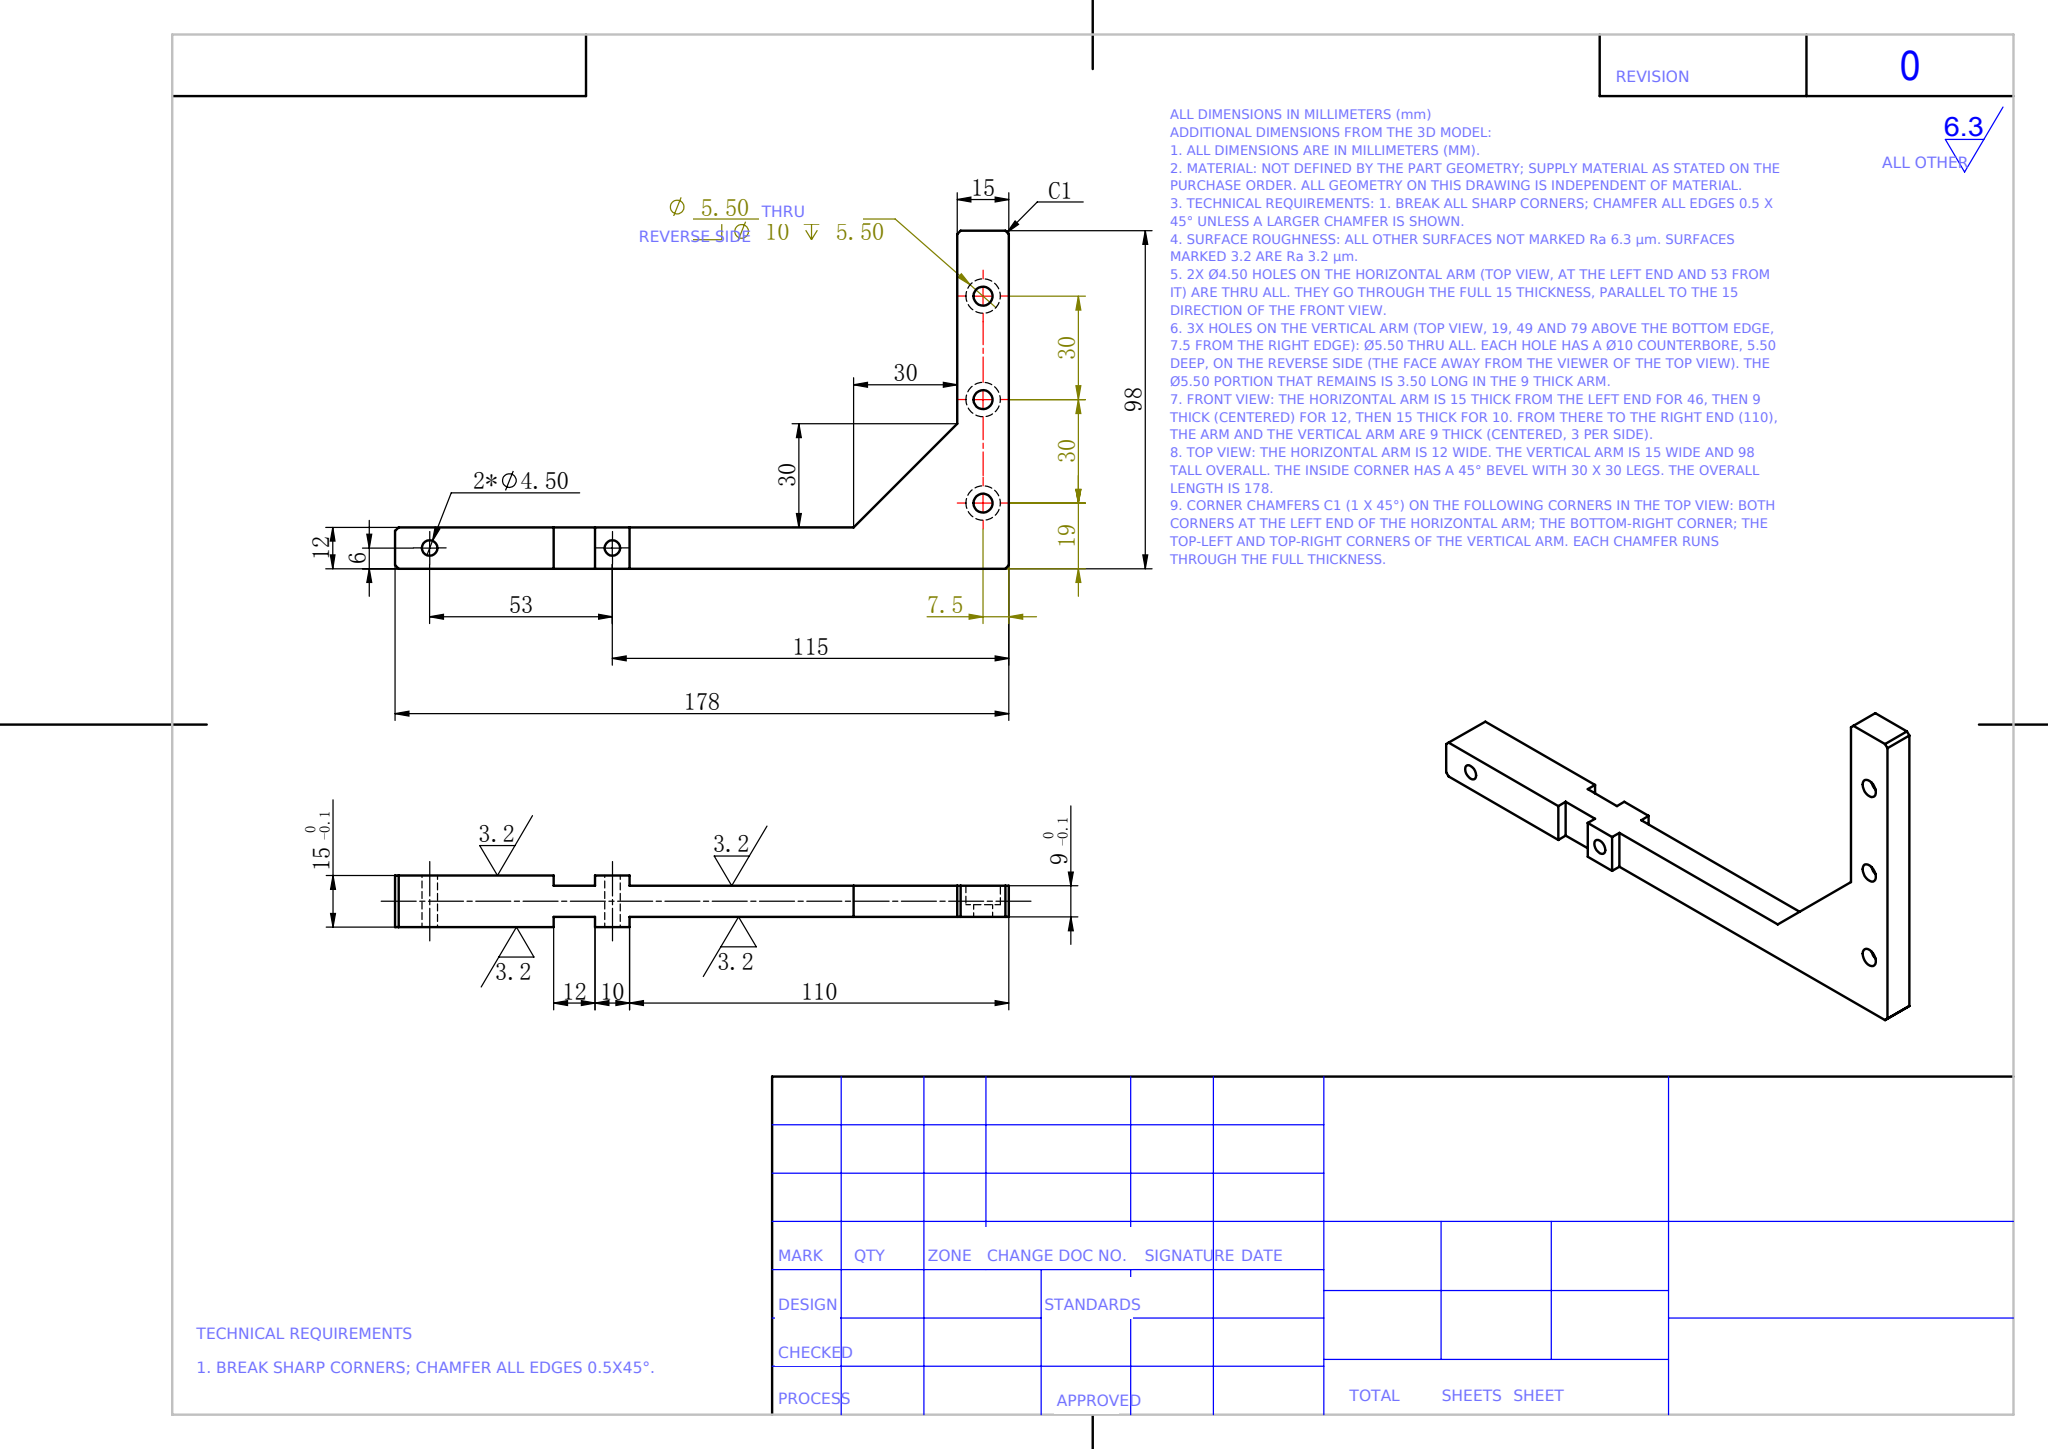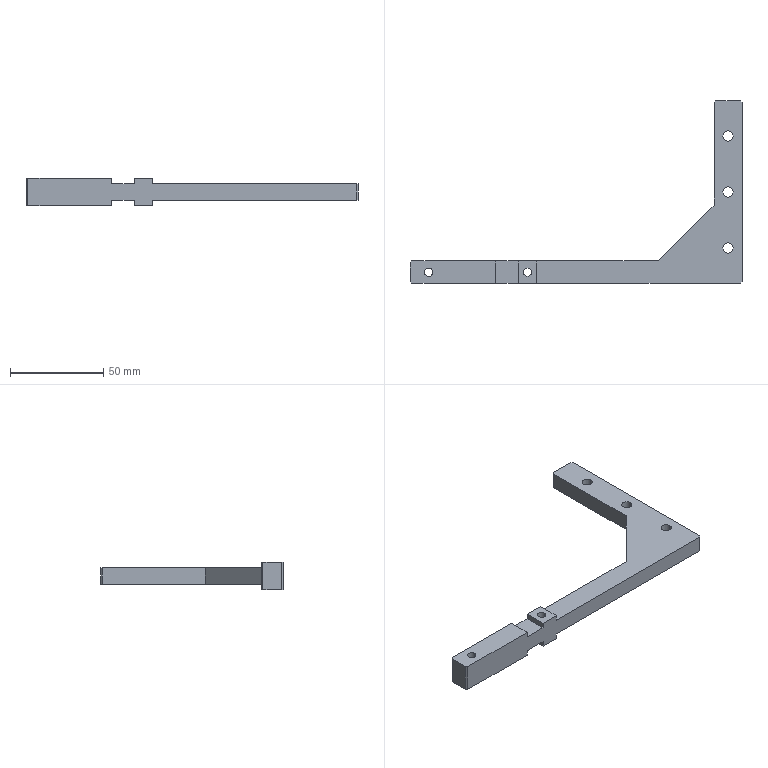Part | NX | mm | 1 solid | 45 faces | box 178 x 98 x 15 mm | volume 36865 mm3 | plane 29 | cylinder 16 | commonest cylinder face diameters 10 x6 5.5 x6 4.5 x4